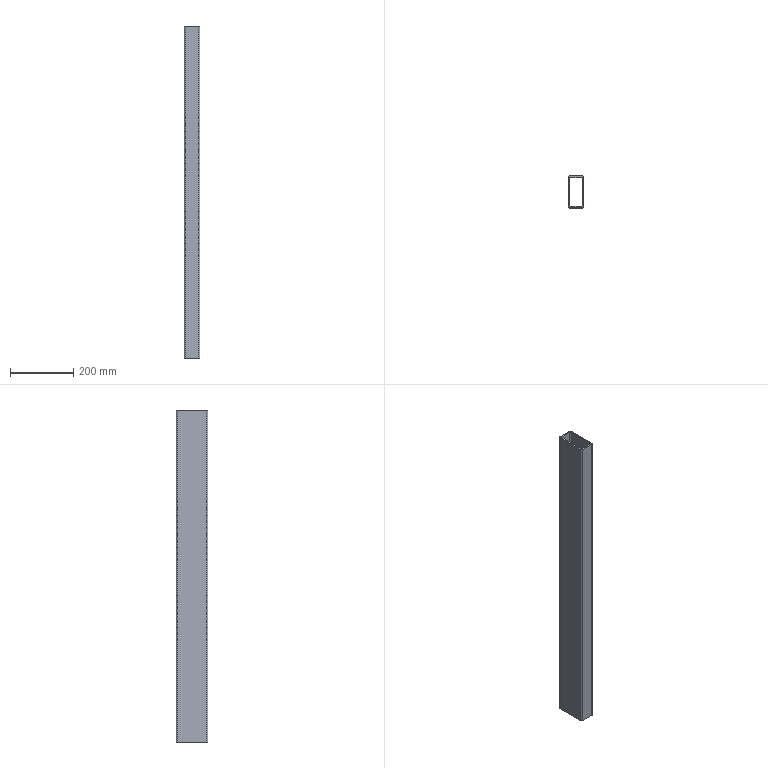Component | NX | BASE_FRAME_RECT_TUBE | 1 solid | 18 faces | volume 1192800 mm3 | plane 10 | cylinder 8 | commonest cylinder face diameters 8 x8